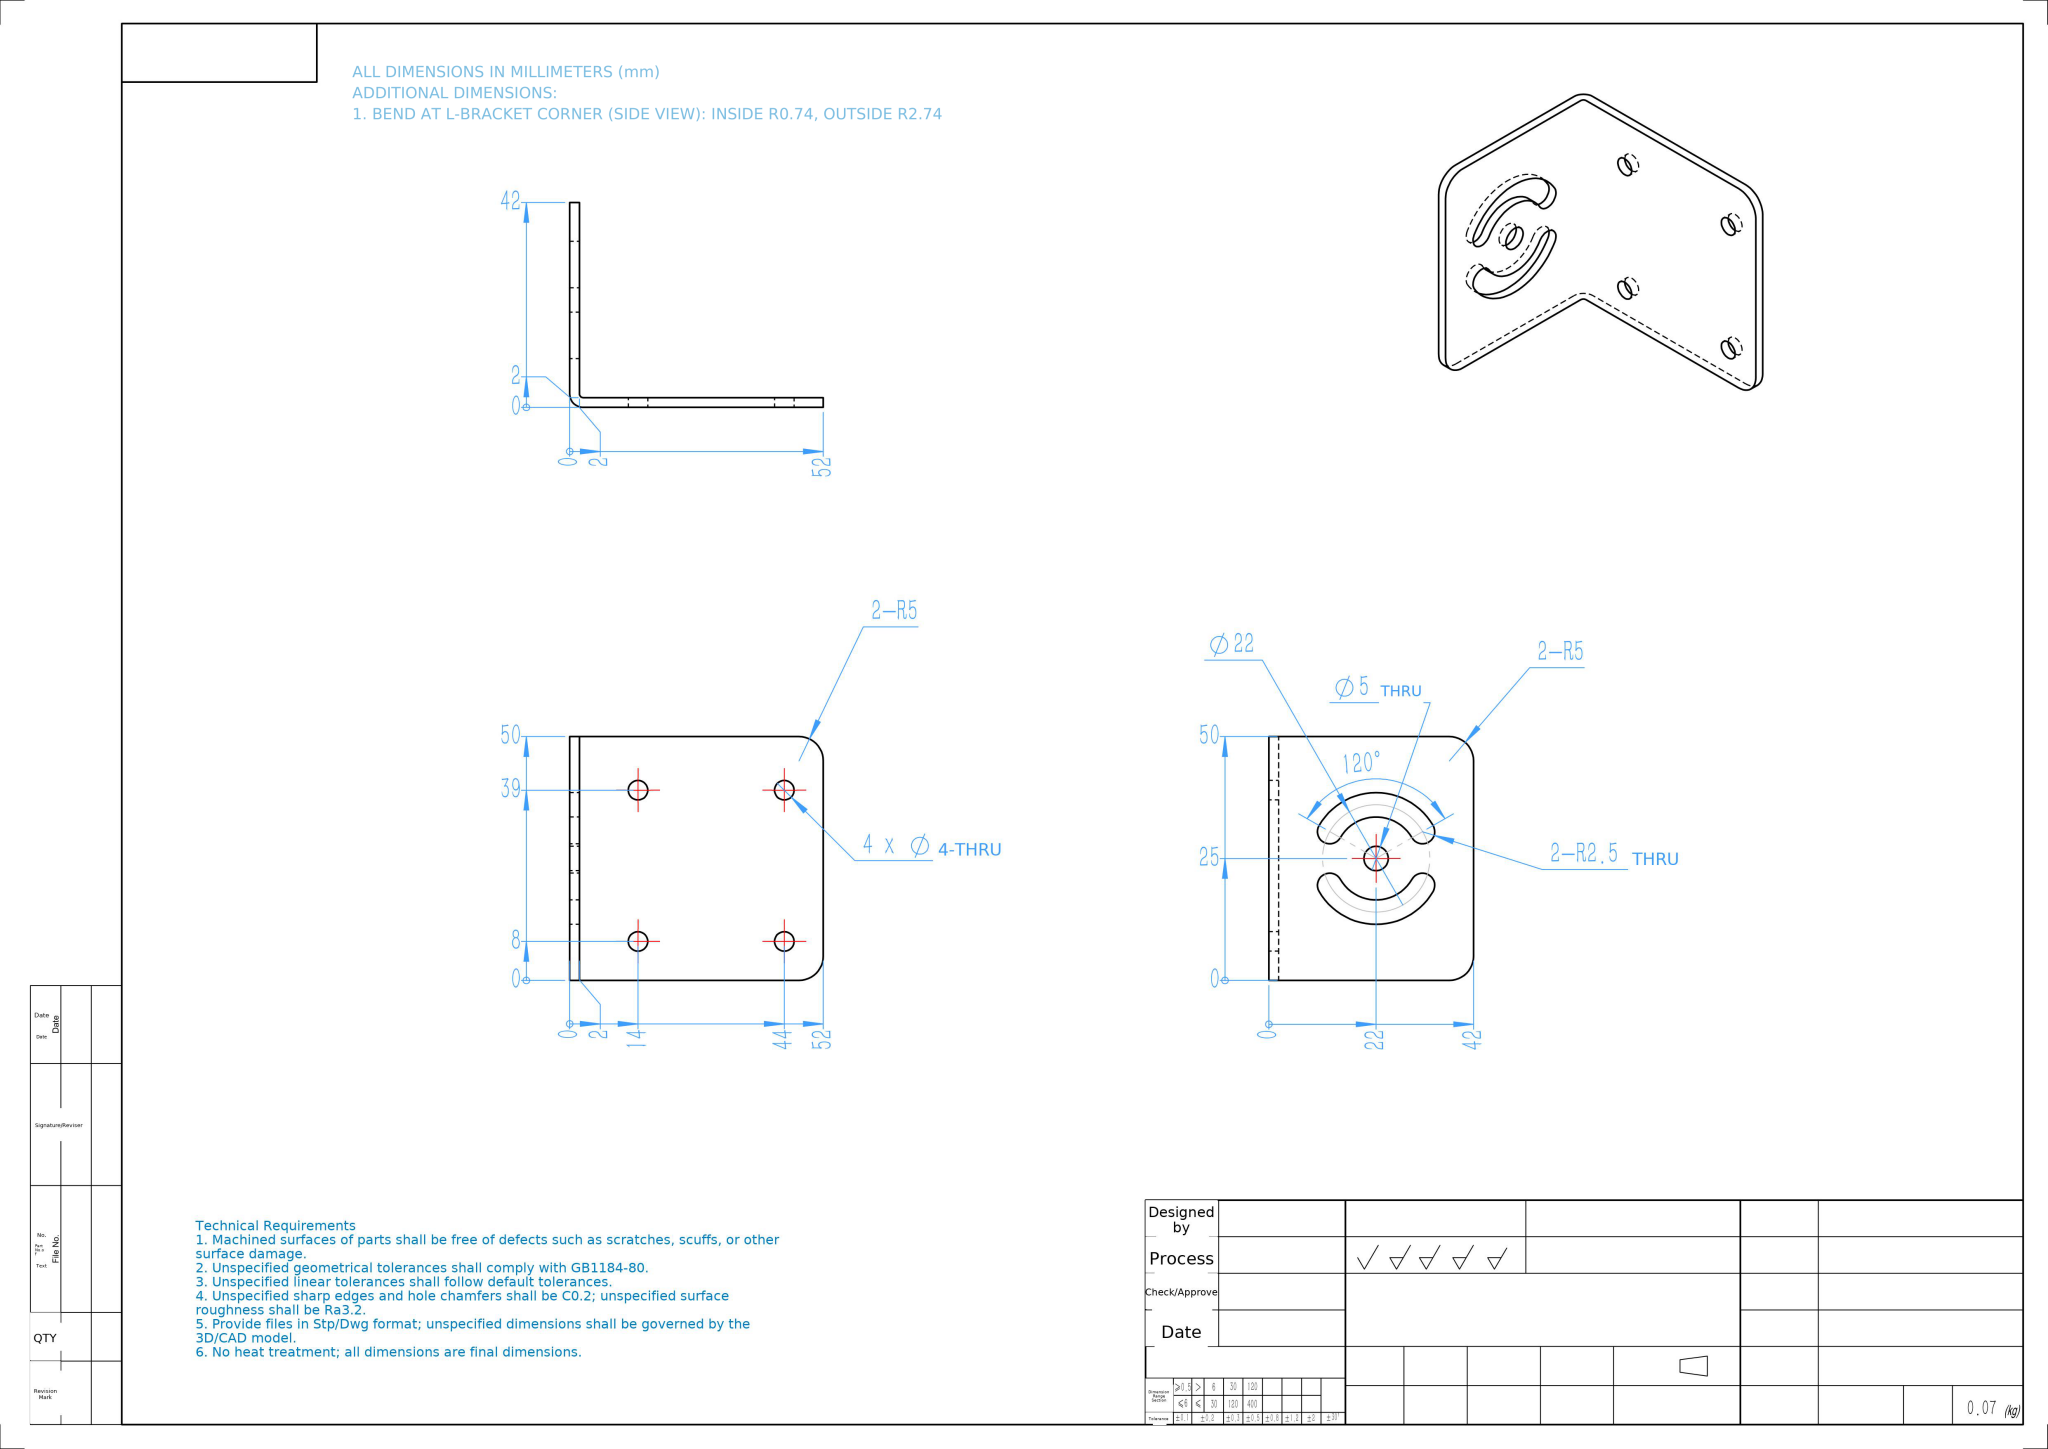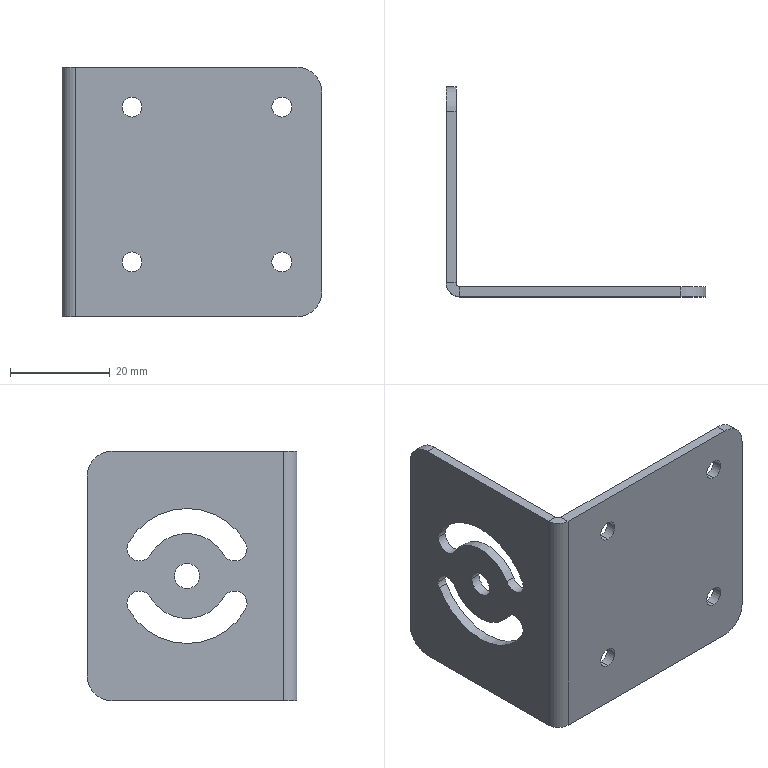Part | NX | mm | 1 solid | 38 faces | box 52 x 42 x 50 mm | volume 8403 mm3 | cylinder 26 | plane 12 | commonest cylinder face diameters 5 x8 4 x8 10 x4 17 x2 27 x2 1.473 x1 5.473 x1